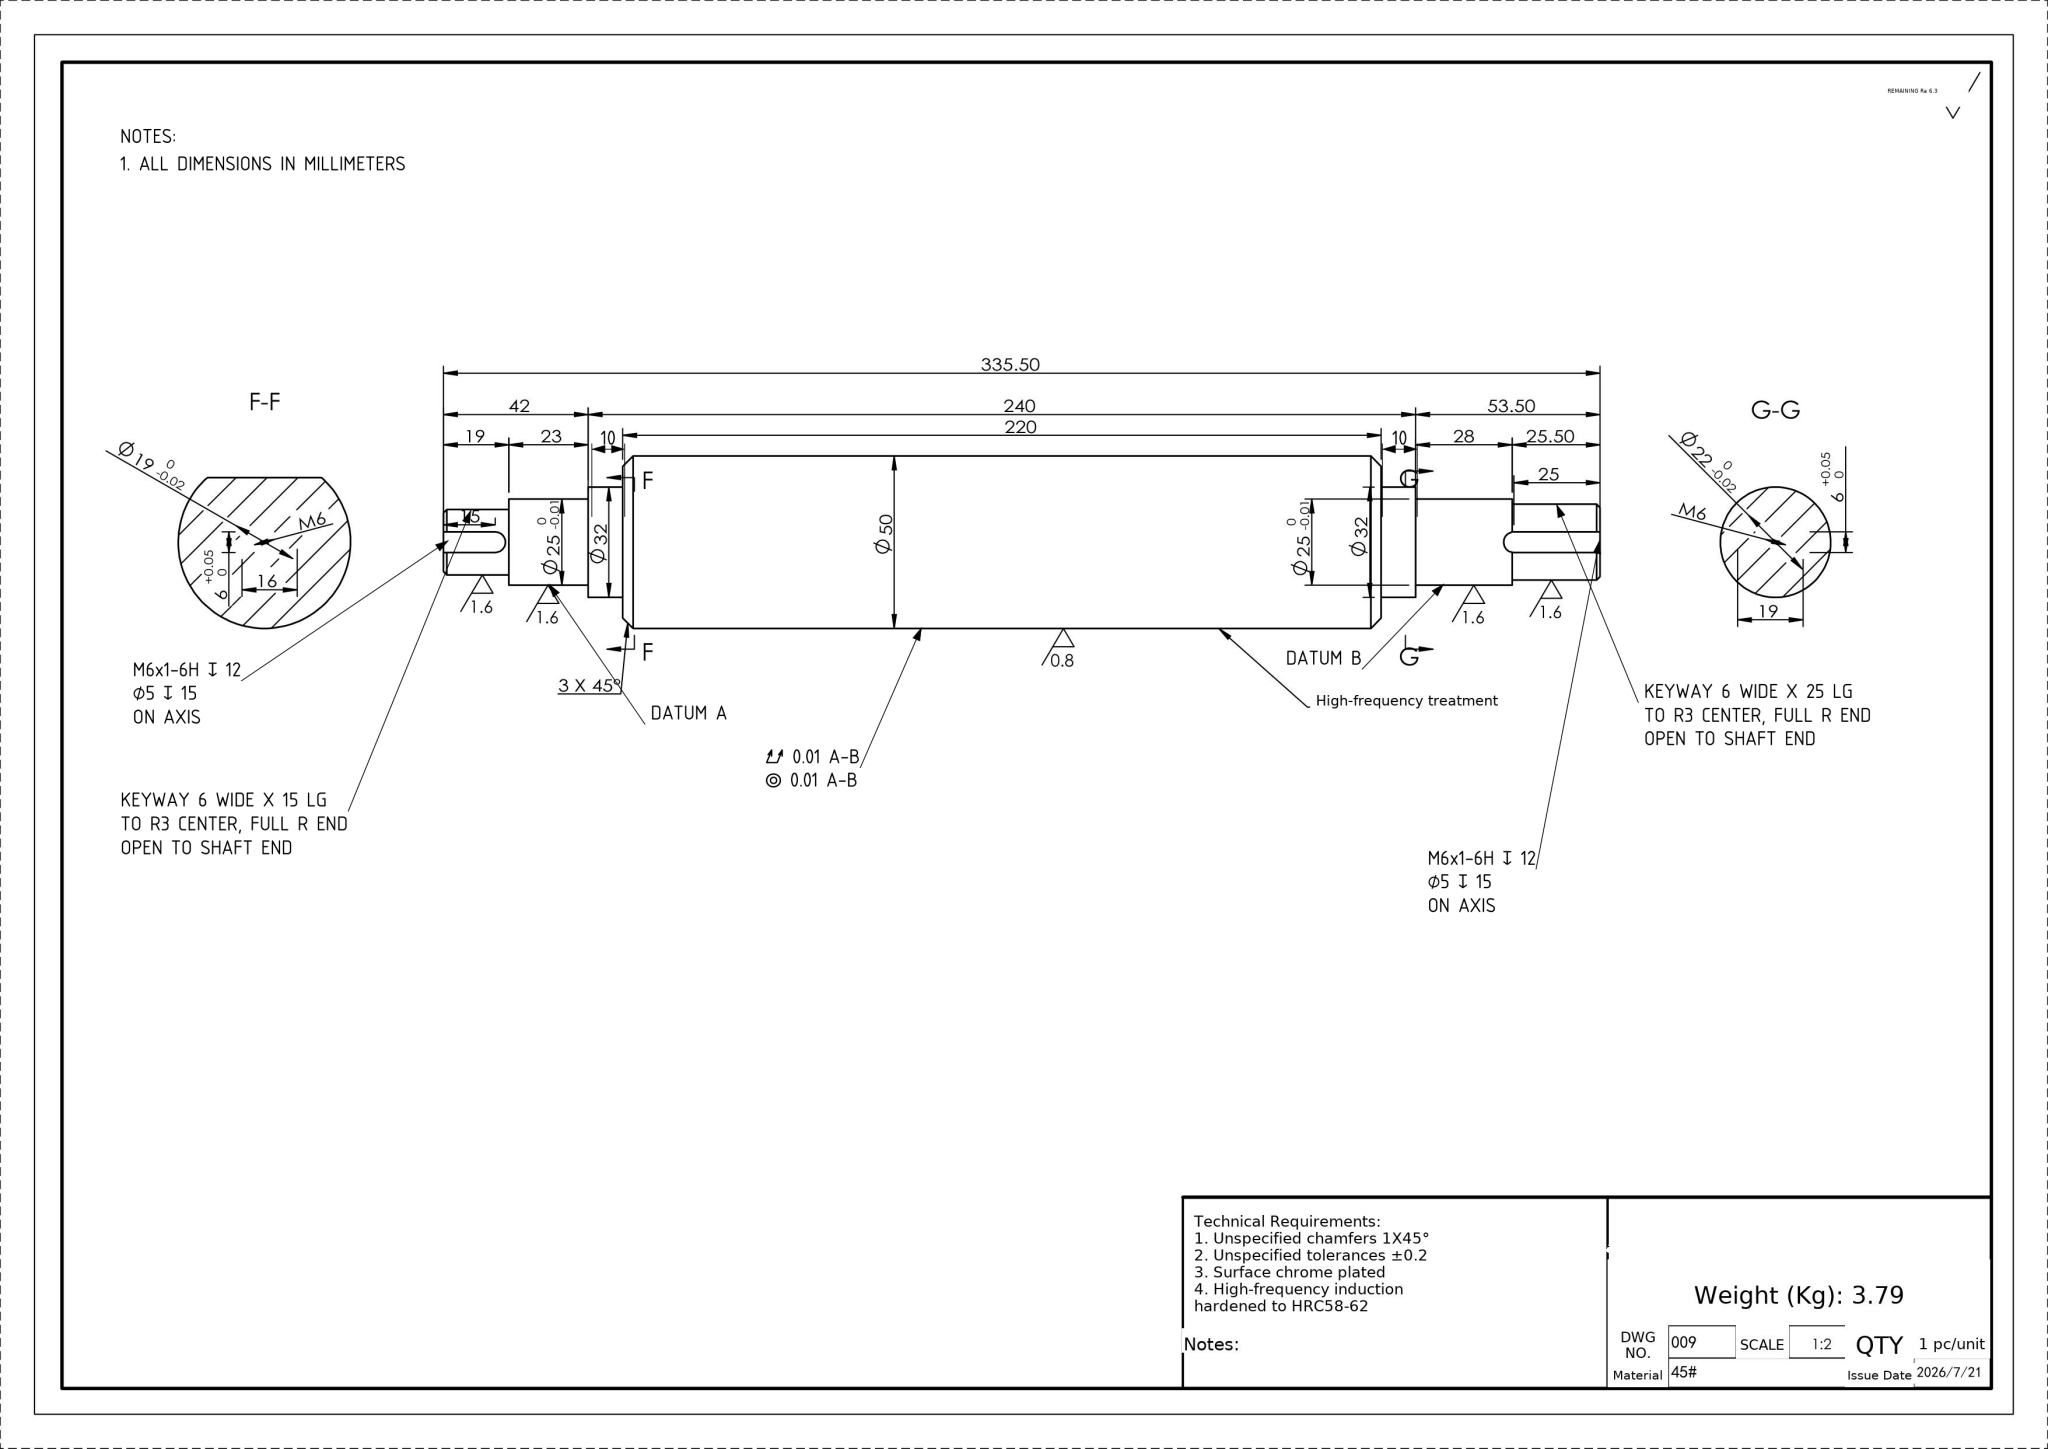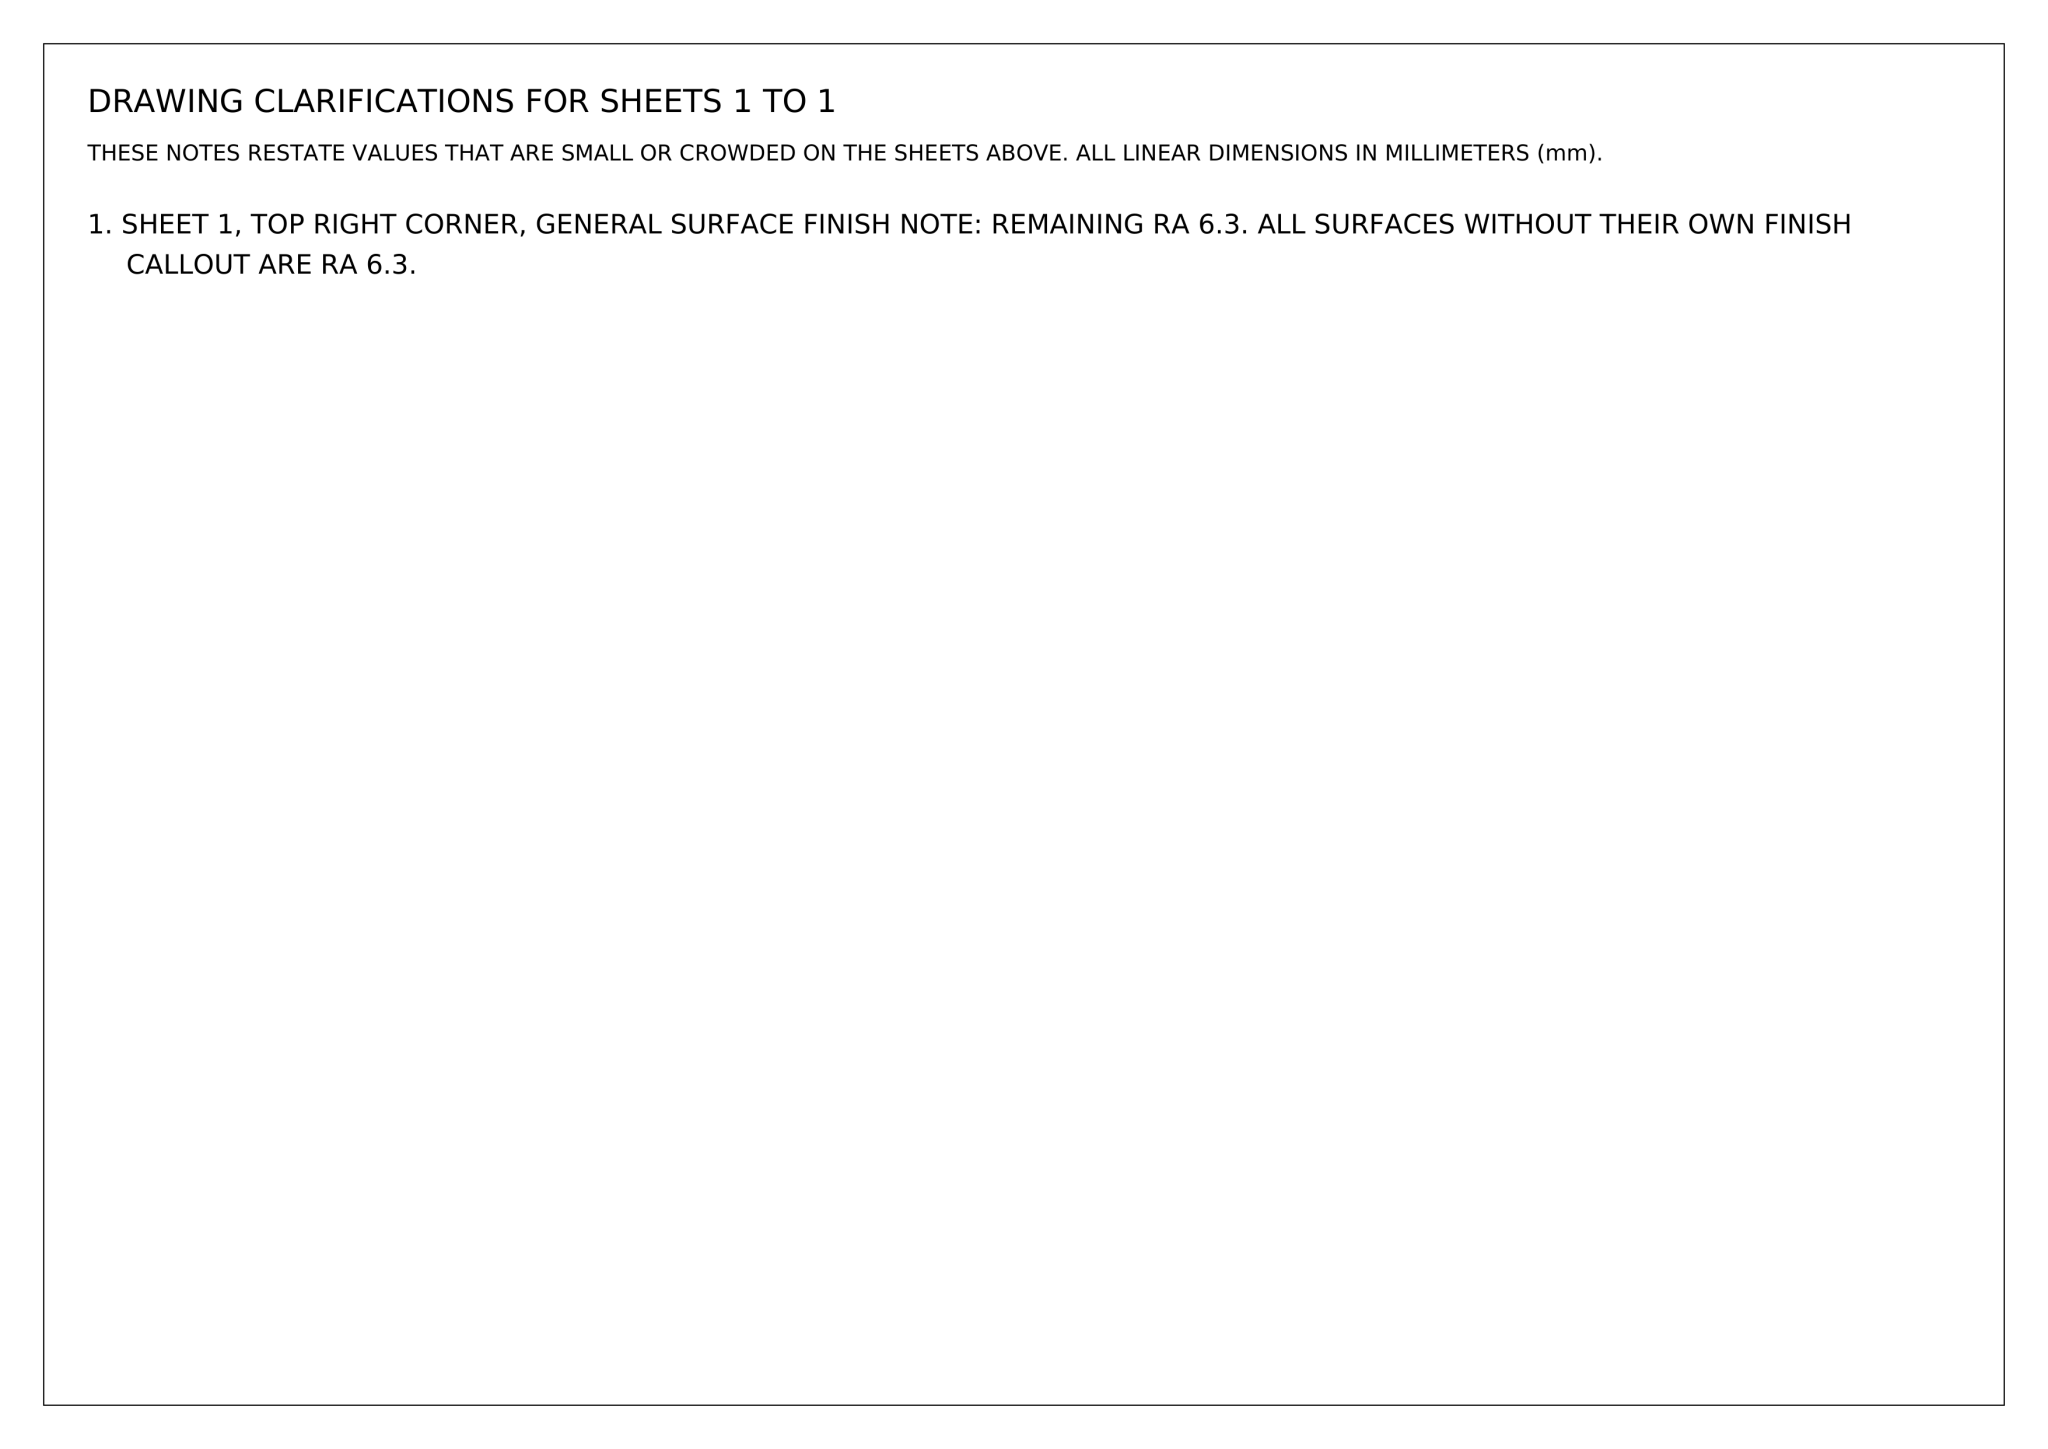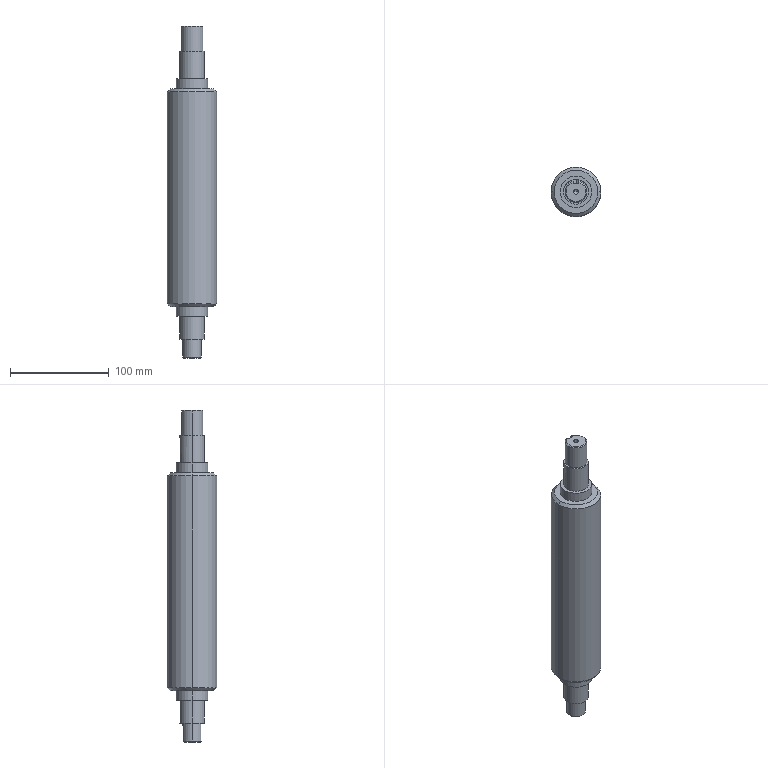Part | NX | mm | 1 solid | 51 faces | box 50 x 50 x 335.5 mm | volume 485285 mm3 | cylinder 23 | cone 14 | plane 14 | commonest cylinder face diameters 6 x4 5 x4 32 x4 25 x4 22 x3 19 x2 50 x2